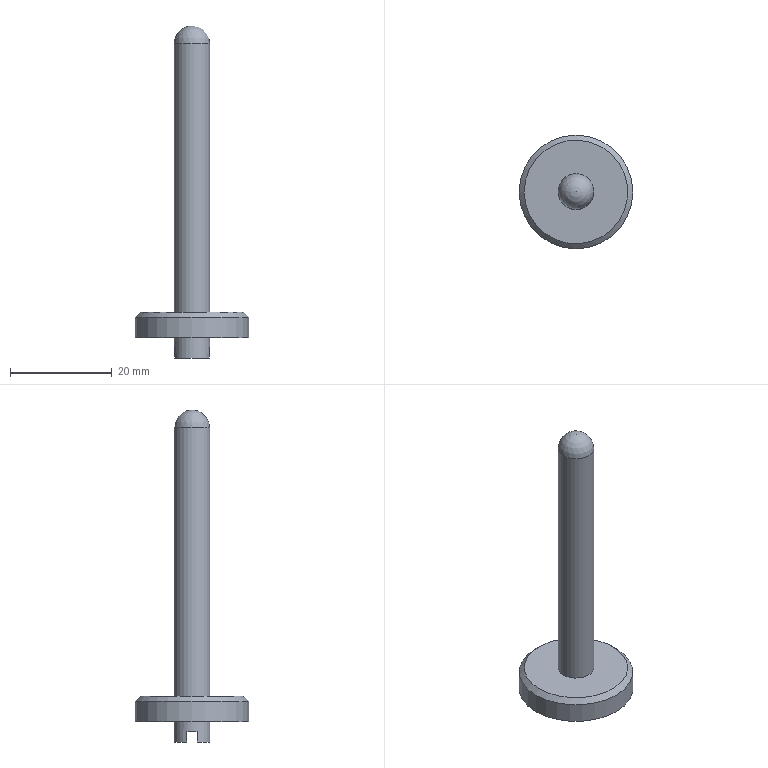Component | NX | VALVE_STEM | 1 solid | 12 faces | box 22.37 x 22.37 x 65.29 mm | volume 4179 mm3 | plane 7 | cylinder 3 | cone 1 | sphere 1 | commonest cylinder face diameters 7 x2 22.369 x1
STEP:
#1=CARTESIAN_POINT('',(0.,0.,0.));
#2=DIRECTION('',(0.,0.,1.));
#3=DIRECTION('',(1.,0.,0.));
#4=AXIS2_PLACEMENT_3D('',#1,#2,#3);
#5=CARTESIAN_POINT('',(-3.354,1.,34.567));
#6=VERTEX_POINT('',#5);
#7=CARTESIAN_POINT('',(3.354,1.,34.567));
#8=VERTEX_POINT('',#7);
#9=CARTESIAN_POINT('',(-8.45,1.,34.567));
#10=DIRECTION('',(1.,0.,0.));
#11=VECTOR('',#10,1.);
#12=LINE('',#9,#11);
#13=CARTESIAN_POINT('',(0.,0.,34.567));
#14=DIRECTION('',(0.,0.,-1.));
#15=DIRECTION('',(-1.,0.,0.));
#16=AXIS2_PLACEMENT_3D('',#13,#14,#15);
#17=PLANE('',#16);
#18=CARTESIAN_POINT('',(8.45,1.));
#19=DIRECTION('',(-1.,0.));
#20=VECTOR('',#19,1.);
#21=LINE('',#18,#20);
#22=(GEOMETRIC_REPRESENTATION_CONTEXT(2)PARAMETRIC_REPRESENTATION_CONTEXT()REPRESENTATION_CONTEXT('',''));
#23=DEFINITIONAL_REPRESENTATION('',(#21),#22);
#24=PCURVE('',#17,#23);
#25=CARTESIAN_POINT('',(-8.45,1.,36.567));
#26=DIRECTION('',(0.,1.,0.));
#27=DIRECTION('',(0.,0.,1.));
#28=AXIS2_PLACEMENT_3D('',#25,#26,#27);
#29=PLANE('',#28);
#30=CARTESIAN_POINT('',(-2.,0.));
#31=DIRECTION('',(0.,1.));
#32=VECTOR('',#31,1.);
#33=LINE('',#30,#32);
#34=(GEOMETRIC_REPRESENTATION_CONTEXT(2)PARAMETRIC_REPRESENTATION_CONTEXT()REPRESENTATION_CONTEXT('',''));
#35=DEFINITIONAL_REPRESENTATION('',(#33),#34);
#36=PCURVE('',#29,#35);
#37=SURFACE_CURVE('',#12,(#24,#36),.PCURVE_S1.);
#38=EDGE_CURVE('',#6,#8,#37,.T.);
#39=ORIENTED_EDGE('',*,*,#38,.F.);
#40=CARTESIAN_POINT('',(0.,0.,34.567));
#41=DIRECTION('',(0.,0.,-1.));
#42=DIRECTION('',(1.,0.,0.));
#43=AXIS2_PLACEMENT_3D('',#40,#41,#42);
#44=CIRCLE('',#43,3.5);
#45=CARTESIAN_POINT('',(0.,0.));
#46=DIRECTION('',(-1.,0.));
#47=AXIS2_PLACEMENT_2D('',#45,#46);
#48=CIRCLE('',#47,3.5);
#49=(GEOMETRIC_REPRESENTATION_CONTEXT(2)PARAMETRIC_REPRESENTATION_CONTEXT()REPRESENTATION_CONTEXT('',''));
#50=DEFINITIONAL_REPRESENTATION('',(#48),#49);
#51=PCURVE('',#17,#50);
#52=CARTESIAN_POINT('',(0.,0.,34.567));
#53=DIRECTION('',(0.,0.,1.));
#54=DIRECTION('',(1.,0.,0.));
#55=AXIS2_PLACEMENT_3D('',#52,#53,#54);
#56=CYLINDRICAL_SURFACE('',#55,3.5);
#57=CARTESIAN_POINT('',(6.283,0.));
#58=DIRECTION('',(-1.,0.));
#59=VECTOR('',#58,1.);
#60=LINE('',#57,#59);
#61=(GEOMETRIC_REPRESENTATION_CONTEXT(2)PARAMETRIC_REPRESENTATION_CONTEXT()REPRESENTATION_CONTEXT('',''));
#62=DEFINITIONAL_REPRESENTATION('',(#60),#61);
#63=PCURVE('',#56,#62);
#64=SURFACE_CURVE('',#44,(#51,#63),.PCURVE_S1.);
#65=EDGE_CURVE('',#6,#8,#64,.T.);
#66=ORIENTED_EDGE('',*,*,#65,.T.);
#67=EDGE_LOOP('',(#39,#66));
#68=FACE_BOUND('',#67,.T.);
#69=ADVANCED_FACE('',(#68),#17,.T.);
#70=CARTESIAN_POINT('',(3.5,0.,38.567));
#71=VERTEX_POINT('',#70);
#72=CARTESIAN_POINT('',(0.,0.,38.567));
#73=DIRECTION('',(0.,0.,-1.));
#74=DIRECTION('',(1.,0.,0.));
#75=AXIS2_PLACEMENT_3D('',#72,#73,#74);
#76=CIRCLE('',#75,3.5);
#77=CARTESIAN_POINT('',(0.,0.,38.567));
#78=DIRECTION('',(0.,0.,1.));
#79=DIRECTION('',(1.,0.,0.));
#80=AXIS2_PLACEMENT_3D('',#77,#78,#79);
#81=PLANE('',#80);
#82=CARTESIAN_POINT('',(3.5,-0.));
#83=CARTESIAN_POINT('',(3.5,-6.062));
#84=CARTESIAN_POINT('',(-1.75,-3.031));
#85=CARTESIAN_POINT('',(-7.,-0.));
#86=CARTESIAN_POINT('',(-1.75,3.031));
#87=CARTESIAN_POINT('',(3.5,6.062));
#88=CARTESIAN_POINT('',(3.5,-0.));
#89=(BOUNDED_CURVE()B_SPLINE_CURVE(2,(#82,#83,#84,#85,#86,#87,#88),.UNSPECIFIED.,.T.,.F.)B_SPLINE_CURVE_WITH_KNOTS((1,2,2,2,2,1),(-2.094,0.,2.094,4.189,6.283,8.378),.UNSPECIFIED.)CURVE()GEOMETRIC_REPRESENTATION_ITEM()RATIONAL_B_SPLINE_CURVE((1.,0.5,1.,0.5,1.,0.5,1.))REPRESENTATION_ITEM(''));
#90=(GEOMETRIC_REPRESENTATION_CONTEXT(2)PARAMETRIC_REPRESENTATION_CONTEXT()REPRESENTATION_CONTEXT('',''));
#91=DEFINITIONAL_REPRESENTATION('',(#89),#90);
#92=PCURVE('',#81,#91);
#93=CARTESIAN_POINT('',(6.283,4.));
#94=DIRECTION('',(-1.,0.));
#95=VECTOR('',#94,1.);
#96=LINE('',#93,#95);
#97=(GEOMETRIC_REPRESENTATION_CONTEXT(2)PARAMETRIC_REPRESENTATION_CONTEXT()REPRESENTATION_CONTEXT('',''));
#98=DEFINITIONAL_REPRESENTATION('',(#96),#97);
#99=PCURVE('',#56,#98);
#100=SURFACE_CURVE('',#76,(#92,#99),.PCURVE_S1.);
#101=EDGE_CURVE('',#71,#71,#100,.T.);
#102=ORIENTED_EDGE('',*,*,#101,.F.);
#103=EDGE_LOOP('',(#102));
#104=FACE_BOUND('',#103,.T.);
#105=CARTESIAN_POINT('',(11.184,0.,38.567));
#106=VERTEX_POINT('',#105);
#107=CARTESIAN_POINT('',(0.,0.,38.567));
#108=DIRECTION('',(0.,0.,1.));
#109=DIRECTION('',(1.,0.,0.));
#110=AXIS2_PLACEMENT_3D('',#107,#108,#109);
#111=CIRCLE('',#110,11.184);
#112=CARTESIAN_POINT('',(0.,-0.));
#113=DIRECTION('',(1.,0.));
#114=AXIS2_PLACEMENT_2D('',#112,#113);
#115=CIRCLE('',#114,11.184);
#116=(GEOMETRIC_REPRESENTATION_CONTEXT(2)PARAMETRIC_REPRESENTATION_CONTEXT()REPRESENTATION_CONTEXT('',''));
#117=DEFINITIONAL_REPRESENTATION('',(#115),#116);
#118=PCURVE('',#81,#117);
#119=CARTESIAN_POINT('',(0.,0.,79.857));
#120=DIRECTION('',(0.,0.,1.));
#121=DIRECTION('',(1.,0.,0.));
#122=AXIS2_PLACEMENT_3D('',#119,#120,#121);
#123=CYLINDRICAL_SURFACE('',#122,11.184);
#124=CARTESIAN_POINT('',(0.,-41.29));
#125=DIRECTION('',(1.,0.));
#126=VECTOR('',#125,1.);
#127=LINE('',#124,#126);
#128=(GEOMETRIC_REPRESENTATION_CONTEXT(2)PARAMETRIC_REPRESENTATION_CONTEXT()REPRESENTATION_CONTEXT('',''));
#129=DEFINITIONAL_REPRESENTATION('',(#127),#128);
#130=PCURVE('',#123,#129);
#131=SURFACE_CURVE('',#111,(#118,#130),.PCURVE_S1.);
#132=EDGE_CURVE('',#106,#106,#131,.T.);
#133=ORIENTED_EDGE('',*,*,#132,.F.);
#134=EDGE_LOOP('',(#133));
#135=FACE_BOUND('',#134,.T.);
#136=ADVANCED_FACE('',(#104,#135),#81,.F.);
#137=CARTESIAN_POINT('',(-11.184,0.,42.567));
#138=VERTEX_POINT('',#137);
#139=CARTESIAN_POINT('',(11.184,0.,42.567));
#140=VERTEX_POINT('',#139);
#141=CARTESIAN_POINT('',(0.,0.,42.567));
#142=DIRECTION('',(0.,0.,-1.));
#143=DIRECTION('',(-1.,0.,0.));
#144=AXIS2_PLACEMENT_3D('',#141,#142,#143);
#145=CIRCLE('',#144,11.184);
#146=CARTESIAN_POINT('',(3.142,-37.29));
#147=DIRECTION('',(-1.,0.));
#148=VECTOR('',#147,1.);
#149=LINE('',#146,#148);
#150=(GEOMETRIC_REPRESENTATION_CONTEXT(2)PARAMETRIC_REPRESENTATION_CONTEXT()REPRESENTATION_CONTEXT('',''));
#151=DEFINITIONAL_REPRESENTATION('',(#149),#150);
#152=PCURVE('',#123,#151);
#153=CARTESIAN_POINT('',(0.,0.,43.567));
#154=DIRECTION('',(0.,0.,-1.));
#155=DIRECTION('',(-1.,0.,0.));
#156=AXIS2_PLACEMENT_3D('',#153,#154,#155);
#157=CONICAL_SURFACE('',#156,10.184,0.7854);
#158=CARTESIAN_POINT('',(0.,1.));
#159=DIRECTION('',(1.,0.));
#160=VECTOR('',#159,1.);
#161=LINE('',#158,#160);
#162=(GEOMETRIC_REPRESENTATION_CONTEXT(2)PARAMETRIC_REPRESENTATION_CONTEXT()REPRESENTATION_CONTEXT('',''));
#163=DEFINITIONAL_REPRESENTATION('',(#161),#162);
#164=PCURVE('',#157,#163);
#165=SURFACE_CURVE('',#145,(#152,#164),.PCURVE_S1.);
#166=EDGE_CURVE('',#138,#140,#165,.T.);
#167=ORIENTED_EDGE('',*,*,#166,.T.);
#168=CARTESIAN_POINT('',(11.184,-0.,38.567));
#169=CARTESIAN_POINT('',(11.184,-0.,42.567));
#170=B_SPLINE_CURVE_WITH_KNOTS('',1,(#168,#169),.UNSPECIFIED.,.F.,.F.,(2,2),(-41.29,-37.29),.PIECEWISE_BEZIER_KNOTS.);
#171=CARTESIAN_POINT('',(0.,0.));
#172=DIRECTION('',(0.,1.));
#173=VECTOR('',#172,1.);
#174=LINE('',#171,#173);
#175=(GEOMETRIC_REPRESENTATION_CONTEXT(2)PARAMETRIC_REPRESENTATION_CONTEXT()REPRESENTATION_CONTEXT('',''));
#176=DEFINITIONAL_REPRESENTATION('',(#174),#175);
#177=PCURVE('',#123,#176);
#178=CARTESIAN_POINT('',(6.283,0.));
#179=DIRECTION('',(0.,1.));
#180=VECTOR('',#179,1.);
#181=LINE('',#178,#180);
#182=(GEOMETRIC_REPRESENTATION_CONTEXT(2)PARAMETRIC_REPRESENTATION_CONTEXT()REPRESENTATION_CONTEXT('',''));
#183=DEFINITIONAL_REPRESENTATION('',(#181),#182);
#184=PCURVE('',#123,#183);
#185=SEAM_CURVE('',#170,(#177,#184),.PCURVE_S1.);
#186=EDGE_CURVE('',#106,#140,#185,.T.);
#187=ORIENTED_EDGE('',*,*,#186,.F.);
#188=ORIENTED_EDGE('',*,*,#132,.T.);
#189=ORIENTED_EDGE('',*,*,#186,.T.);
#190=CARTESIAN_POINT('',(0.,0.,42.567));
#191=DIRECTION('',(0.,0.,-1.));
#192=DIRECTION('',(-1.,0.,0.));
#193=AXIS2_PLACEMENT_3D('',#190,#191,#192);
#194=CIRCLE('',#193,11.184);
#195=CARTESIAN_POINT('',(9.425,-37.29));
#196=DIRECTION('',(-1.,0.));
#197=VECTOR('',#196,1.);
#198=LINE('',#195,#197);
#199=(GEOMETRIC_REPRESENTATION_CONTEXT(2)PARAMETRIC_REPRESENTATION_CONTEXT()REPRESENTATION_CONTEXT('',''));
#200=DEFINITIONAL_REPRESENTATION('',(#198),#199);
#201=PCURVE('',#123,#200);
#202=CARTESIAN_POINT('',(0.,1.));
#203=DIRECTION('',(1.,0.));
#204=VECTOR('',#203,1.);
#205=LINE('',#202,#204);
#206=(GEOMETRIC_REPRESENTATION_CONTEXT(2)PARAMETRIC_REPRESENTATION_CONTEXT()REPRESENTATION_CONTEXT('',''));
#207=DEFINITIONAL_REPRESENTATION('',(#205),#206);
#208=PCURVE('',#157,#207);
#209=SURFACE_CURVE('',#194,(#201,#208),.PCURVE_S1.);
#210=EDGE_CURVE('',#140,#138,#209,.T.);
#211=ORIENTED_EDGE('',*,*,#210,.T.);
#212=EDGE_LOOP('',(#167,#187,#188,#189,#211));
#213=FACE_BOUND('',#212,.T.);
#214=ADVANCED_FACE('',(#213),#123,.T.);
#215=CARTESIAN_POINT('',(-10.184,0.,43.567));
#216=VERTEX_POINT('',#215);
#217=CARTESIAN_POINT('',(0.,0.,43.567));
#218=DIRECTION('',(0.,0.,1.));
#219=DIRECTION('',(-1.,0.,0.));
#220=AXIS2_PLACEMENT_3D('',#217,#218,#219);
#221=CIRCLE('',#220,10.184);
#222=CARTESIAN_POINT('',(0.,11.184,43.567));
#223=DIRECTION('',(0.,0.,-1.));
#224=DIRECTION('',(-1.,0.,0.));
#225=AXIS2_PLACEMENT_3D('',#222,#223,#224);
#226=PLANE('',#225);
#227=CARTESIAN_POINT('',(10.184,-11.184));
#228=CARTESIAN_POINT('',(10.184,-28.824));
#229=CARTESIAN_POINT('',(-5.092,-20.004));
#230=CARTESIAN_POINT('',(-20.369,-11.184));
#231=CARTESIAN_POINT('',(-5.092,-2.364));
#232=CARTESIAN_POINT('',(10.184,6.455));
#233=CARTESIAN_POINT('',(10.184,-11.184));
#234=(BOUNDED_CURVE()B_SPLINE_CURVE(2,(#227,#228,#229,#230,#231,#232,#233),.UNSPECIFIED.,.T.,.F.)B_SPLINE_CURVE_WITH_KNOTS((1,2,2,2,2,1),(-2.094,0.,2.094,4.189,6.283,8.378),.UNSPECIFIED.)CURVE()GEOMETRIC_REPRESENTATION_ITEM()RATIONAL_B_SPLINE_CURVE((1.,0.5,1.,0.5,1.,0.5,1.))REPRESENTATION_ITEM(''));
#235=(GEOMETRIC_REPRESENTATION_CONTEXT(2)PARAMETRIC_REPRESENTATION_CONTEXT()REPRESENTATION_CONTEXT('',''));
#236=DEFINITIONAL_REPRESENTATION('',(#234),#235);
#237=PCURVE('',#226,#236);
#238=CARTESIAN_POINT('',(6.283,0.));
#239=DIRECTION('',(-1.,0.));
#240=VECTOR('',#239,1.);
#241=LINE('',#238,#240);
#242=(GEOMETRIC_REPRESENTATION_CONTEXT(2)PARAMETRIC_REPRESENTATION_CONTEXT()REPRESENTATION_CONTEXT('',''));
#243=DEFINITIONAL_REPRESENTATION('',(#241),#242);
#244=PCURVE('',#157,#243);
#245=SURFACE_CURVE('',#221,(#237,#244),.PCURVE_S1.);
#246=EDGE_CURVE('',#216,#216,#245,.T.);
#247=ORIENTED_EDGE('',*,*,#246,.T.);
#248=EDGE_LOOP('',(#247));
#249=FACE_BOUND('',#248,.T.);
#250=CARTESIAN_POINT('',(3.5,0.,43.567));
#251=VERTEX_POINT('',#250);
#252=CARTESIAN_POINT('',(0.,0.,43.567));
#253=DIRECTION('',(0.,0.,1.));
#254=DIRECTION('',(1.,0.,0.));
#255=AXIS2_PLACEMENT_3D('',#252,#253,#254);
#256=CIRCLE('',#255,3.5);
#257=CARTESIAN_POINT('',(-3.5,-11.184));
#258=CARTESIAN_POINT('',(-3.5,-5.122));
#259=CARTESIAN_POINT('',(1.75,-8.153));
#260=CARTESIAN_POINT('',(7.,-11.184));
#261=CARTESIAN_POINT('',(1.75,-14.215));
#262=CARTESIAN_POINT('',(-3.5,-17.246));
#263=CARTESIAN_POINT('',(-3.5,-11.184));
#264=(BOUNDED_CURVE()B_SPLINE_CURVE(2,(#257,#258,#259,#260,#261,#262,#263),.UNSPECIFIED.,.T.,.F.)B_SPLINE_CURVE_WITH_KNOTS((1,2,2,2,2,1),(-2.094,0.,2.094,4.189,6.283,8.378),.UNSPECIFIED.)CURVE()GEOMETRIC_REPRESENTATION_ITEM()RATIONAL_B_SPLINE_CURVE((1.,0.5,1.,0.5,1.,0.5,1.))REPRESENTATION_ITEM(''));
#265=(GEOMETRIC_REPRESENTATION_CONTEXT(2)PARAMETRIC_REPRESENTATION_CONTEXT()REPRESENTATION_CONTEXT('',''));
#266=DEFINITIONAL_REPRESENTATION('',(#264),#265);
#267=PCURVE('',#226,#266);
#268=CARTESIAN_POINT('',(0.,0.,79.857));
#269=DIRECTION('',(0.,0.,1.));
#270=DIRECTION('',(1.,0.,0.));
#271=AXIS2_PLACEMENT_3D('',#268,#269,#270);
#272=CYLINDRICAL_SURFACE('',#271,3.5);
#273=CARTESIAN_POINT('',(0.,-36.29));
#274=DIRECTION('',(1.,0.));
#275=VECTOR('',#274,1.);
#276=LINE('',#273,#275);
#277=(GEOMETRIC_REPRESENTATION_CONTEXT(2)PARAMETRIC_REPRESENTATION_CONTEXT()REPRESENTATION_CONTEXT('',''));
#278=DEFINITIONAL_REPRESENTATION('',(#276),#277);
#279=PCURVE('',#272,#278);
#280=SURFACE_CURVE('',#256,(#267,#279),.PCURVE_S1.);
#281=EDGE_CURVE('',#251,#251,#280,.T.);
#282=ORIENTED_EDGE('',*,*,#281,.F.);
#283=EDGE_LOOP('',(#282));
#284=FACE_BOUND('',#283,.T.);
#285=ADVANCED_FACE('',(#249,#284),#226,.F.);
#286=CARTESIAN_POINT('',(3.5,0.,96.357));
#287=VERTEX_POINT('',#286);
#288=CARTESIAN_POINT('',(-3.5,0.,96.357));
#289=VERTEX_POINT('',#288);
#290=CARTESIAN_POINT('',(0.,0.,96.357));
#291=DIRECTION('',(0.,0.,-1.));
#292=DIRECTION('',(1.,0.,0.));
#293=AXIS2_PLACEMENT_3D('',#290,#291,#292);
#294=CIRCLE('',#293,3.5);
#295=CARTESIAN_POINT('',(6.283,16.5));
#296=DIRECTION('',(-1.,0.));
#297=VECTOR('',#296,1.);
#298=LINE('',#295,#297);
#299=(GEOMETRIC_REPRESENTATION_CONTEXT(2)PARAMETRIC_REPRESENTATION_CONTEXT()REPRESENTATION_CONTEXT('',''));
#300=DEFINITIONAL_REPRESENTATION('',(#298),#299);
#301=PCURVE('',#272,#300);
#302=CARTESIAN_POINT('',(0.,0.,96.357));
#303=DIRECTION('',(-0.,0.,-1.));
#304=DIRECTION('',(-1.,0.,0.));
#305=AXIS2_PLACEMENT_3D('',#302,#303,#304);
#306=SPHERICAL_SURFACE('',#305,3.5);
#307=CARTESIAN_POINT('',(3.142,0.));
#308=CARTESIAN_POINT('',(3.237,0.));
#309=CARTESIAN_POINT('',(3.427,0.));
#310=CARTESIAN_POINT('',(3.713,0.));
#311=CARTESIAN_POINT('',(3.998,0.));
#312=CARTESIAN_POINT('',(4.284,0.));
#313=CARTESIAN_POINT('',(4.57,0.));
#314=CARTESIAN_POINT('',(4.855,0.));
#315=CARTESIAN_POINT('',(5.141,0.));
#316=CARTESIAN_POINT('',(5.426,0.));
#317=CARTESIAN_POINT('',(5.712,0.));
#318=CARTESIAN_POINT('',(5.998,0.));
#319=CARTESIAN_POINT('',(6.283,0.));
#320=CARTESIAN_POINT('',(6.569,0.));
#321=CARTESIAN_POINT('',(6.854,0.));
#322=CARTESIAN_POINT('',(7.14,0.));
#323=CARTESIAN_POINT('',(7.426,0.));
#324=CARTESIAN_POINT('',(7.711,0.));
#325=CARTESIAN_POINT('',(7.997,0.));
#326=CARTESIAN_POINT('',(8.282,0.));
#327=CARTESIAN_POINT('',(8.568,0.));
#328=CARTESIAN_POINT('',(8.854,0.));
#329=CARTESIAN_POINT('',(9.139,0.));
#330=CARTESIAN_POINT('',(9.33,0.));
#331=CARTESIAN_POINT('',(9.425,0.));
#332=B_SPLINE_CURVE_WITH_KNOTS('',3,(#307,#308,#309,#310,#311,#312,#313,#314,#315,#316,#317,#318,#319,#320,#321,#322,#323,#324,#325,#326,#327,#328,#329,#330,#331),.UNSPECIFIED.,.F.,.F.,(4,1,1,1,1,1,1,1,1,1,1,1,1,1,1,1,1,1,1,1,1,1,4),(0.,0.2856,0.5712,0.8568,1.142,1.428,1.714,1.999,2.285,2.57,2.856,3.142,3.427,3.713,3.998,4.284,4.57,4.855,5.141,5.426,5.712,5.998,6.283),.QUASI_UNIFORM_KNOTS.);
#333=(GEOMETRIC_REPRESENTATION_CONTEXT(2)PARAMETRIC_REPRESENTATION_CONTEXT()REPRESENTATION_CONTEXT('',''));
#334=DEFINITIONAL_REPRESENTATION('',(#332),#333);
#335=PCURVE('',#306,#334);
#336=SURFACE_CURVE('',#294,(#301,#335),.PCURVE_S1.);
#337=EDGE_CURVE('',#287,#289,#336,.T.);
#338=ORIENTED_EDGE('',*,*,#337,.T.);
#339=CARTESIAN_POINT('',(0.,0.,96.357));
#340=DIRECTION('',(0.,0.,-1.));
#341=DIRECTION('',(1.,0.,0.));
#342=AXIS2_PLACEMENT_3D('',#339,#340,#341);
#343=CIRCLE('',#342,3.5);
#344=CARTESIAN_POINT('',(6.283,16.5));
#345=DIRECTION('',(-1.,0.));
#346=VECTOR('',#345,1.);
#347=LINE('',#344,#346);
#348=(GEOMETRIC_REPRESENTATION_CONTEXT(2)PARAMETRIC_REPRESENTATION_CONTEXT()REPRESENTATION_CONTEXT('',''));
#349=DEFINITIONAL_REPRESENTATION('',(#347),#348);
#350=PCURVE('',#272,#349);
#351=CARTESIAN_POINT('',(-3.142,0.));
#352=CARTESIAN_POINT('',(-3.046,0.));
#353=CARTESIAN_POINT('',(-2.856,0.));
#354=CARTESIAN_POINT('',(-2.57,0.));
#355=CARTESIAN_POINT('',(-2.285,0.));
#356=CARTESIAN_POINT('',(-1.999,0.));
#357=CARTESIAN_POINT('',(-1.714,0.));
#358=CARTESIAN_POINT('',(-1.428,0.));
#359=CARTESIAN_POINT('',(-1.142,0.));
#360=CARTESIAN_POINT('',(-0.8568,0.));
#361=CARTESIAN_POINT('',(-0.5712,0.));
#362=CARTESIAN_POINT('',(-0.2856,0.));
#363=CARTESIAN_POINT('',(0.,0.));
#364=CARTESIAN_POINT('',(0.2856,0.));
#365=CARTESIAN_POINT('',(0.5712,0.));
#366=CARTESIAN_POINT('',(0.8568,0.));
#367=CARTESIAN_POINT('',(1.142,0.));
#368=CARTESIAN_POINT('',(1.428,0.));
#369=CARTESIAN_POINT('',(1.714,0.));
#370=CARTESIAN_POINT('',(1.999,0.));
#371=CARTESIAN_POINT('',(2.285,0.));
#372=CARTESIAN_POINT('',(2.57,0.));
#373=CARTESIAN_POINT('',(2.856,0.));
#374=CARTESIAN_POINT('',(3.046,0.));
#375=CARTESIAN_POINT('',(3.142,0.));
#376=B_SPLINE_CURVE_WITH_KNOTS('',3,(#351,#352,#353,#354,#355,#356,#357,#358,#359,#360,#361,#362,#363,#364,#365,#366,#367,#368,#369,#370,#371,#372,#373,#374,#375),.UNSPECIFIED.,.F.,.F.,(4,1,1,1,1,1,1,1,1,1,1,1,1,1,1,1,1,1,1,1,1,1,4),(0.,0.2856,0.5712,0.8568,1.142,1.428,1.714,1.999,2.285,2.57,2.856,3.142,3.427,3.713,3.998,4.284,4.57,4.855,5.141,5.426,5.712,5.998,6.283),.QUASI_UNIFORM_KNOTS.);
#377=(GEOMETRIC_REPRESENTATION_CONTEXT(2)PARAMETRIC_REPRESENTATION_CONTEXT()REPRESENTATION_CONTEXT('',''));
#378=DEFINITIONAL_REPRESENTATION('',(#376),#377);
#379=PCURVE('',#306,#378);
#380=SURFACE_CURVE('',#343,(#350,#379),.PCURVE_S1.);
#381=EDGE_CURVE('',#289,#287,#380,.T.);
#382=ORIENTED_EDGE('',*,*,#381,.T.);
#383=CARTESIAN_POINT('',(3.5,-0.,43.567));
#384=CARTESIAN_POINT('',(3.5,-0.,96.357));
#385=B_SPLINE_CURVE_WITH_KNOTS('',1,(#383,#384),.UNSPECIFIED.,.F.,.F.,(2,2),(-36.29,16.5),.PIECEWISE_BEZIER_KNOTS.);
#386=CARTESIAN_POINT('',(0.,0.));
#387=DIRECTION('',(0.,1.));
#388=VECTOR('',#387,1.);
#389=LINE('',#386,#388);
#390=(GEOMETRIC_REPRESENTATION_CONTEXT(2)PARAMETRIC_REPRESENTATION_CONTEXT()REPRESENTATION_CONTEXT('',''));
#391=DEFINITIONAL_REPRESENTATION('',(#389),#390);
#392=PCURVE('',#272,#391);
#393=CARTESIAN_POINT('',(6.283,0.));
#394=DIRECTION('',(0.,1.));
#395=VECTOR('',#394,1.);
#396=LINE('',#393,#395);
#397=(GEOMETRIC_REPRESENTATION_CONTEXT(2)PARAMETRIC_REPRESENTATION_CONTEXT()REPRESENTATION_CONTEXT('',''));
#398=DEFINITIONAL_REPRESENTATION('',(#396),#397);
#399=PCURVE('',#272,#398);
#400=SEAM_CURVE('',#385,(#392,#399),.PCURVE_S1.);
#401=EDGE_CURVE('',#251,#287,#400,.T.);
#402=ORIENTED_EDGE('',*,*,#401,.F.);
#403=ORIENTED_EDGE('',*,*,#281,.T.);
#404=ORIENTED_EDGE('',*,*,#401,.T.);
#405=EDGE_LOOP('',(#338,#382,#402,#403,#404));
#406=FACE_BOUND('',#405,.T.);
#407=ADVANCED_FACE('',(#406),#272,.T.);
#408=ORIENTED_EDGE('',*,*,#166,.F.);
#409=CARTESIAN_POINT('',(-10.184,-0.,43.567));
#410=CARTESIAN_POINT('',(-11.184,-0.,42.567));
#411=B_SPLINE_CURVE_WITH_KNOTS('',1,(#409,#410),.UNSPECIFIED.,.F.,.F.,(2,2),(0.,1.414),.PIECEWISE_BEZIER_KNOTS.);
#412=CARTESIAN_POINT('',(0.,0.));
#413=DIRECTION('',(0.,1.));
#414=VECTOR('',#413,1.);
#415=LINE('',#412,#414);
#416=(GEOMETRIC_REPRESENTATION_CONTEXT(2)PARAMETRIC_REPRESENTATION_CONTEXT()REPRESENTATION_CONTEXT('',''));
#417=DEFINITIONAL_REPRESENTATION('',(#415),#416);
#418=PCURVE('',#157,#417);
#419=CARTESIAN_POINT('',(6.283,0.));
#420=DIRECTION('',(0.,1.));
#421=VECTOR('',#420,1.);
#422=LINE('',#419,#421);
#423=(GEOMETRIC_REPRESENTATION_CONTEXT(2)PARAMETRIC_REPRESENTATION_CONTEXT()REPRESENTATION_CONTEXT('',''));
#424=DEFINITIONAL_REPRESENTATION('',(#422),#423);
#425=PCURVE('',#157,#424);
#426=SEAM_CURVE('',#411,(#418,#425),.PCURVE_S1.);
#427=EDGE_CURVE('',#216,#138,#426,.T.);
#428=ORIENTED_EDGE('',*,*,#427,.F.);
#429=ORIENTED_EDGE('',*,*,#246,.F.);
#430=ORIENTED_EDGE('',*,*,#427,.T.);
#431=ORIENTED_EDGE('',*,*,#210,.F.);
#432=EDGE_LOOP('',(#408,#428,#429,#430,#431));
#433=FACE_BOUND('',#432,.T.);
#434=ADVANCED_FACE('',(#433),#157,.T.);
#435=CARTESIAN_POINT('',(3.5,0.,36.567));
#436=VERTEX_POINT('',#435);
#437=CARTESIAN_POINT('',(3.354,-1.,36.567));
#438=VERTEX_POINT('',#437);
#439=CARTESIAN_POINT('',(0.,0.,36.567));
#440=DIRECTION('',(0.,0.,-1.));
#441=DIRECTION('',(-1.,0.,0.));
#442=AXIS2_PLACEMENT_3D('',#439,#440,#441);
#443=CIRCLE('',#442,3.5);
#444=CARTESIAN_POINT('',(9.425,2.));
#445=DIRECTION('',(-1.,0.));
#446=VECTOR('',#445,1.);
#447=LINE('',#444,#446);
#448=(GEOMETRIC_REPRESENTATION_CONTEXT(2)PARAMETRIC_REPRESENTATION_CONTEXT()REPRESENTATION_CONTEXT('',''));
#449=DEFINITIONAL_REPRESENTATION('',(#447),#448);
#450=PCURVE('',#56,#449);
#451=CARTESIAN_POINT('',(0.,0.,36.567));
#452=DIRECTION('',(0.,0.,-1.));
#453=DIRECTION('',(-1.,0.,0.));
#454=AXIS2_PLACEMENT_3D('',#451,#452,#453);
#455=PLANE('',#454);
#456=CARTESIAN_POINT('',(0.,0.));
#457=DIRECTION('',(1.,0.));
#458=AXIS2_PLACEMENT_2D('',#456,#457);
#459=CIRCLE('',#458,3.5);
#460=(GEOMETRIC_REPRESENTATION_CONTEXT(2)PARAMETRIC_REPRESENTATION_CONTEXT()REPRESENTATION_CONTEXT('',''));
#461=DEFINITIONAL_REPRESENTATION('',(#459),#460);
#462=PCURVE('',#455,#461);
#463=SURFACE_CURVE('',#443,(#450,#462),.PCURVE_S1.);
#464=EDGE_CURVE('',#436,#438,#463,.T.);
#465=ORIENTED_EDGE('',*,*,#464,.F.);
#466=CARTESIAN_POINT('',(3.5,0.,36.567));
#467=CARTESIAN_POINT('',(3.5,0.,38.567));
#468=B_SPLINE_CURVE_WITH_KNOTS('',1,(#466,#467),.UNSPECIFIED.,.F.,.F.,(2,2),(2.,4.),.PIECEWISE_BEZIER_KNOTS.);
#469=CARTESIAN_POINT('',(6.283,0.));
#470=DIRECTION('',(0.,1.));
#471=VECTOR('',#470,1.);
#472=LINE('',#469,#471);
#473=(GEOMETRIC_REPRESENTATION_CONTEXT(2)PARAMETRIC_REPRESENTATION_CONTEXT()REPRESENTATION_CONTEXT('',''));
#474=DEFINITIONAL_REPRESENTATION('',(#472),#473);
#475=PCURVE('',#56,#474);
#476=CARTESIAN_POINT('',(0.,0.));
#477=DIRECTION('',(0.,1.));
#478=VECTOR('',#477,1.);
#479=LINE('',#476,#478);
#480=(GEOMETRIC_REPRESENTATION_CONTEXT(2)PARAMETRIC_REPRESENTATION_CONTEXT()REPRESENTATION_CONTEXT('',''));
#481=DEFINITIONAL_REPRESENTATION('',(#479),#480);
#482=PCURVE('',#56,#481);
#483=SEAM_CURVE('',#468,(#475,#482),.PCURVE_S1.);
#484=EDGE_CURVE('',#436,#71,#483,.T.);
#485=ORIENTED_EDGE('',*,*,#484,.T.);
#486=ORIENTED_EDGE('',*,*,#101,.T.);
#487=ORIENTED_EDGE('',*,*,#484,.F.);
#488=CARTESIAN_POINT('',(3.354,1.,36.567));
#489=VERTEX_POINT('',#488);
#490=CARTESIAN_POINT('',(0.,0.,36.567));
#491=DIRECTION('',(0.,0.,-1.));
#492=DIRECTION('',(-1.,0.,0.));
#493=AXIS2_PLACEMENT_3D('',#490,#491,#492);
#494=CIRCLE('',#493,3.5);
#495=CARTESIAN_POINT('',(3.142,2.));
#496=DIRECTION('',(-1.,0.));
#497=VECTOR('',#496,1.);
#498=LINE('',#495,#497);
#499=(GEOMETRIC_REPRESENTATION_CONTEXT(2)PARAMETRIC_REPRESENTATION_CONTEXT()REPRESENTATION_CONTEXT('',''));
#500=DEFINITIONAL_REPRESENTATION('',(#498),#499);
#501=PCURVE('',#56,#500);
#502=CARTESIAN_POINT('',(0.,0.));
#503=DIRECTION('',(1.,0.));
#504=AXIS2_PLACEMENT_2D('',#502,#503);
#505=CIRCLE('',#504,3.5);
#506=(GEOMETRIC_REPRESENTATION_CONTEXT(2)PARAMETRIC_REPRESENTATION_CONTEXT()REPRESENTATION_CONTEXT('',''));
#507=DEFINITIONAL_REPRESENTATION('',(#505),#506);
#508=PCURVE('',#455,#507);
#509=SURFACE_CURVE('',#494,(#501,#508),.PCURVE_S1.);
#510=EDGE_CURVE('',#489,#436,#509,.T.);
#511=ORIENTED_EDGE('',*,*,#510,.F.);
#512=CARTESIAN_POINT('',(3.354,1.,34.567));
#513=DIRECTION('',(0.,0.,-1.));
#514=VECTOR('',#513,1.);
#515=LINE('',#512,#514);
#516=CARTESIAN_POINT('',(0.2898,0.));
#517=DIRECTION('',(0.,-1.));
#518=VECTOR('',#517,1.);
#519=LINE('',#516,#518);
#520=(GEOMETRIC_REPRESENTATION_CONTEXT(2)PARAMETRIC_REPRESENTATION_CONTEXT()REPRESENTATION_CONTEXT('',''));
#521=DEFINITIONAL_REPRESENTATION('',(#519),#520);
#522=PCURVE('',#56,#521);
#523=CARTESIAN_POINT('',(-2.,11.804));
#524=DIRECTION('',(-1.,0.));
#525=VECTOR('',#524,1.);
#526=LINE('',#523,#525);
#527=(GEOMETRIC_REPRESENTATION_CONTEXT(2)PARAMETRIC_REPRESENTATION_CONTEXT()REPRESENTATION_CONTEXT('',''));
#528=DEFINITIONAL_REPRESENTATION('',(#526),#527);
#529=PCURVE('',#29,#528);
#530=SURFACE_CURVE('',#515,(#522,#529),.PCURVE_S1.);
#531=EDGE_CURVE('',#489,#8,#530,.T.);
#532=ORIENTED_EDGE('',*,*,#531,.T.);
#533=ORIENTED_EDGE('',*,*,#65,.F.);
#534=CARTESIAN_POINT('',(-3.354,1.,36.567));
#535=VERTEX_POINT('',#534);
#536=CARTESIAN_POINT('',(-3.354,1.,34.567));
#537=DIRECTION('',(0.,0.,1.));
#538=VECTOR('',#537,1.);
#539=LINE('',#536,#538);
#540=CARTESIAN_POINT('',(2.852,0.));
#541=DIRECTION('',(0.,1.));
#542=VECTOR('',#541,1.);
#543=LINE('',#540,#542);
#544=(GEOMETRIC_REPRESENTATION_CONTEXT(2)PARAMETRIC_REPRESENTATION_CONTEXT()REPRESENTATION_CONTEXT('',''));
#545=DEFINITIONAL_REPRESENTATION('',(#543),#544);
#546=PCURVE('',#56,#545);
#547=CARTESIAN_POINT('',(-2.,5.096));
#548=DIRECTION('',(1.,0.));
#549=VECTOR('',#548,1.);
#550=LINE('',#547,#549);
#551=(GEOMETRIC_REPRESENTATION_CONTEXT(2)PARAMETRIC_REPRESENTATION_CONTEXT()REPRESENTATION_CONTEXT('',''));
#552=DEFINITIONAL_REPRESENTATION('',(#550),#551);
#553=PCURVE('',#29,#552);
#554=SURFACE_CURVE('',#539,(#546,#553),.PCURVE_S1.);
#555=EDGE_CURVE('',#6,#535,#554,.T.);
#556=ORIENTED_EDGE('',*,*,#555,.T.);
#557=CARTESIAN_POINT('',(-3.354,-1.,36.567));
#558=VERTEX_POINT('',#557);
#559=CARTESIAN_POINT('',(0.,0.,36.567));
#560=DIRECTION('',(0.,0.,-1.));
#561=DIRECTION('',(-1.,0.,0.));
#562=AXIS2_PLACEMENT_3D('',#559,#560,#561);
#563=CIRCLE('',#562,3.5);
#564=CARTESIAN_POINT('',(9.425,2.));
#565=DIRECTION('',(-1.,0.));
#566=VECTOR('',#565,1.);
#567=LINE('',#564,#566);
#568=(GEOMETRIC_REPRESENTATION_CONTEXT(2)PARAMETRIC_REPRESENTATION_CONTEXT()REPRESENTATION_CONTEXT('',''));
#569=DEFINITIONAL_REPRESENTATION('',(#567),#568);
#570=PCURVE('',#56,#569);
#571=CARTESIAN_POINT('',(0.,0.));
#572=DIRECTION('',(1.,0.));
#573=AXIS2_PLACEMENT_2D('',#571,#572);
#574=CIRCLE('',#573,3.5);
#575=(GEOMETRIC_REPRESENTATION_CONTEXT(2)PARAMETRIC_REPRESENTATION_CONTEXT()REPRESENTATION_CONTEXT('',''));
#576=DEFINITIONAL_REPRESENTATION('',(#574),#575);
#577=PCURVE('',#455,#576);
#578=SURFACE_CURVE('',#563,(#570,#577),.PCURVE_S1.);
#579=EDGE_CURVE('',#558,#535,#578,.T.);
#580=ORIENTED_EDGE('',*,*,#579,.F.);
#581=CARTESIAN_POINT('',(-3.354,-1.,34.567));
#582=VERTEX_POINT('',#581);
#583=CARTESIAN_POINT('',(-3.354,-1.,34.567));
#584=DIRECTION('',(0.,0.,-1.));
#585=VECTOR('',#584,1.);
#586=LINE('',#583,#585);
#587=CARTESIAN_POINT('',(3.431,0.));
#588=DIRECTION('',(0.,-1.));
#589=VECTOR('',#588,1.);
#590=LINE('',#587,#589);
#591=(GEOMETRIC_REPRESENTATION_CONTEXT(2)PARAMETRIC_REPRESENTATION_CONTEXT()REPRESENTATION_CONTEXT('',''));
#592=DEFINITIONAL_REPRESENTATION('',(#590),#591);
#593=PCURVE('',#56,#592);
#594=CARTESIAN_POINT('',(8.45,-1.,36.567));
#595=DIRECTION('',(0.,-1.,0.));
#596=DIRECTION('',(0.,0.,-1.));
#597=AXIS2_PLACEMENT_3D('',#594,#595,#596);
#598=PLANE('',#597);
#599=CARTESIAN_POINT('',(2.,-11.804));
#600=DIRECTION('',(1.,0.));
#601=VECTOR('',#600,1.);
#602=LINE('',#599,#601);
#603=(GEOMETRIC_REPRESENTATION_CONTEXT(2)PARAMETRIC_REPRESENTATION_CONTEXT()REPRESENTATION_CONTEXT('',''));
#604=DEFINITIONAL_REPRESENTATION('',(#602),#603);
#605=PCURVE('',#598,#604);
#606=SURFACE_CURVE('',#586,(#593,#605),.PCURVE_S1.);
#607=EDGE_CURVE('',#558,#582,#606,.T.);
#608=ORIENTED_EDGE('',*,*,#607,.T.);
#609=CARTESIAN_POINT('',(3.354,-1.,34.567));
#610=VERTEX_POINT('',#609);
#611=CARTESIAN_POINT('',(0.,0.,34.567));
#612=DIRECTION('',(0.,0.,-1.));
#613=DIRECTION('',(1.,0.,0.));
#614=AXIS2_PLACEMENT_3D('',#611,#612,#613);
#615=CIRCLE('',#614,3.5);
#616=CARTESIAN_POINT('',(6.283,0.));
#617=DIRECTION('',(-1.,0.));
#618=VECTOR('',#617,1.);
#619=LINE('',#616,#618);
#620=(GEOMETRIC_REPRESENTATION_CONTEXT(2)PARAMETRIC_REPRESENTATION_CONTEXT()REPRESENTATION_CONTEXT('',''));
#621=DEFINITIONAL_REPRESENTATION('',(#619),#620);
#622=PCURVE('',#56,#621);
#623=CARTESIAN_POINT('',(0.,0.,34.567));
#624=DIRECTION('',(0.,0.,-1.));
#625=DIRECTION('',(-1.,0.,0.));
#626=AXIS2_PLACEMENT_3D('',#623,#624,#625);
#627=PLANE('',#626);
#628=CARTESIAN_POINT('',(0.,0.));
#629=DIRECTION('',(-1.,0.));
#630=AXIS2_PLACEMENT_2D('',#628,#629);
#631=CIRCLE('',#630,3.5);
#632=(GEOMETRIC_REPRESENTATION_CONTEXT(2)PARAMETRIC_REPRESENTATION_CONTEXT()REPRESENTATION_CONTEXT('',''));
#633=DEFINITIONAL_REPRESENTATION('',(#631),#632);
#634=PCURVE('',#627,#633);
#635=SURFACE_CURVE('',#615,(#622,#634),.PCURVE_S1.);
#636=EDGE_CURVE('',#610,#582,#635,.T.);
#637=ORIENTED_EDGE('',*,*,#636,.F.);
#638=CARTESIAN_POINT('',(3.354,-1.,34.567));
#639=DIRECTION('',(0.,0.,1.));
#640=VECTOR('',#639,1.);
#641=LINE('',#638,#640);
#642=CARTESIAN_POINT('',(5.993,0.));
#643=DIRECTION('',(0.,1.));
#644=VECTOR('',#643,1.);
#645=LINE('',#642,#644);
#646=(GEOMETRIC_REPRESENTATION_CONTEXT(2)PARAMETRIC_REPRESENTATION_CONTEXT()REPRESENTATION_CONTEXT('',''));
#647=DEFINITIONAL_REPRESENTATION('',(#645),#646);
#648=PCURVE('',#56,#647);
#649=CARTESIAN_POINT('',(2.,-5.096));
#650=DIRECTION('',(-1.,0.));
#651=VECTOR('',#650,1.);
#652=LINE('',#649,#651);
#653=(GEOMETRIC_REPRESENTATION_CONTEXT(2)PARAMETRIC_REPRESENTATION_CONTEXT()REPRESENTATION_CONTEXT('',''));
#654=DEFINITIONAL_REPRESENTATION('',(#652),#653);
#655=PCURVE('',#598,#654);
#656=SURFACE_CURVE('',#641,(#648,#655),.PCURVE_S1.);
#657=EDGE_CURVE('',#610,#438,#656,.T.);
#658=ORIENTED_EDGE('',*,*,#657,.T.);
#659=EDGE_LOOP('',(#465,#485,#486,#487,#511,#532,#533,#556,#580,#608,#637,#658));
#660=FACE_BOUND('',#659,.T.);
#661=ADVANCED_FACE('',(#660),#56,.T.);
#662=CARTESIAN_POINT('',(8.45,-1.,34.567));
#663=DIRECTION('',(-1.,0.,0.));
#664=VECTOR('',#663,1.);
#665=LINE('',#662,#664);
#666=CARTESIAN_POINT('',(-8.45,-1.));
#667=DIRECTION('',(1.,0.));
#668=VECTOR('',#667,1.);
#669=LINE('',#666,#668);
#670=(GEOMETRIC_REPRESENTATION_CONTEXT(2)PARAMETRIC_REPRESENTATION_CONTEXT()REPRESENTATION_CONTEXT('',''));
#671=DEFINITIONAL_REPRESENTATION('',(#669),#670);
#672=PCURVE('',#627,#671);
#673=CARTESIAN_POINT('',(2.,0.));
#674=DIRECTION('',(0.,-1.));
#675=VECTOR('',#674,1.);
#676=LINE('',#673,#675);
#677=(GEOMETRIC_REPRESENTATION_CONTEXT(2)PARAMETRIC_REPRESENTATION_CONTEXT()REPRESENTATION_CONTEXT('',''));
#678=DEFINITIONAL_REPRESENTATION('',(#676),#677);
#679=PCURVE('',#598,#678);
#680=SURFACE_CURVE('',#665,(#672,#679),.PCURVE_S1.);
#681=EDGE_CURVE('',#610,#582,#680,.T.);
#682=ORIENTED_EDGE('',*,*,#681,.F.);
#683=ORIENTED_EDGE('',*,*,#636,.T.);
#684=EDGE_LOOP('',(#682,#683));
#685=FACE_BOUND('',#684,.T.);
#686=ADVANCED_FACE('',(#685),#627,.T.);
#687=ORIENTED_EDGE('',*,*,#510,.T.);
#688=ORIENTED_EDGE('',*,*,#464,.T.);
#689=CARTESIAN_POINT('',(8.45,-1.,36.567));
#690=DIRECTION('',(1.,0.,0.));
#691=VECTOR('',#690,1.);
#692=LINE('',#689,#691);
#693=CARTESIAN_POINT('',(-8.45,-1.));
#694=DIRECTION('',(-1.,0.));
#695=VECTOR('',#694,1.);
#696=LINE('',#693,#695);
#697=(GEOMETRIC_REPRESENTATION_CONTEXT(2)PARAMETRIC_REPRESENTATION_CONTEXT()REPRESENTATION_CONTEXT('',''));
#698=DEFINITIONAL_REPRESENTATION('',(#696),#697);
#699=PCURVE('',#455,#698);
#700=CARTESIAN_POINT('',(0.,0.));
#701=DIRECTION('',(0.,1.));
#702=VECTOR('',#701,1.);
#703=LINE('',#700,#702);
#704=(GEOMETRIC_REPRESENTATION_CONTEXT(2)PARAMETRIC_REPRESENTATION_CONTEXT()REPRESENTATION_CONTEXT('',''));
#705=DEFINITIONAL_REPRESENTATION('',(#703),#704);
#706=PCURVE('',#598,#705);
#707=SURFACE_CURVE('',#692,(#699,#706),.PCURVE_S1.);
#708=EDGE_CURVE('',#558,#438,#707,.T.);
#709=ORIENTED_EDGE('',*,*,#708,.F.);
#710=ORIENTED_EDGE('',*,*,#579,.T.);
#711=CARTESIAN_POINT('',(-8.45,1.,36.567));
#712=DIRECTION('',(-1.,0.,0.));
#713=VECTOR('',#712,1.);
#714=LINE('',#711,#713);
#715=CARTESIAN_POINT('',(8.45,1.));
#716=DIRECTION('',(1.,0.));
#717=VECTOR('',#716,1.);
#718=LINE('',#715,#717);
#719=(GEOMETRIC_REPRESENTATION_CONTEXT(2)PARAMETRIC_REPRESENTATION_CONTEXT()REPRESENTATION_CONTEXT('',''));
#720=DEFINITIONAL_REPRESENTATION('',(#718),#719);
#721=PCURVE('',#455,#720);
#722=CARTESIAN_POINT('',(0.,0.));
#723=DIRECTION('',(0.,-1.));
#724=VECTOR('',#723,1.);
#725=LINE('',#722,#724);
#726=(GEOMETRIC_REPRESENTATION_CONTEXT(2)PARAMETRIC_REPRESENTATION_CONTEXT()REPRESENTATION_CONTEXT('',''));
#727=DEFINITIONAL_REPRESENTATION('',(#725),#726);
#728=PCURVE('',#29,#727);
#729=SURFACE_CURVE('',#714,(#721,#728),.PCURVE_S1.);
#730=EDGE_CURVE('',#489,#535,#729,.T.);
#731=ORIENTED_EDGE('',*,*,#730,.F.);
#732=EDGE_LOOP('',(#687,#688,#709,#710,#731));
#733=FACE_BOUND('',#732,.T.);
#734=ADVANCED_FACE('',(#733),#455,.T.);
#735=ORIENTED_EDGE('',*,*,#38,.T.);
#736=ORIENTED_EDGE('',*,*,#531,.F.);
#737=ORIENTED_EDGE('',*,*,#730,.T.);
#738=ORIENTED_EDGE('',*,*,#555,.F.);
#739=EDGE_LOOP('',(#735,#736,#737,#738));
#740=FACE_BOUND('',#739,.T.);
#741=ADVANCED_FACE('',(#740),#29,.F.);
#742=ORIENTED_EDGE('',*,*,#681,.T.);
#743=ORIENTED_EDGE('',*,*,#607,.F.);
#744=ORIENTED_EDGE('',*,*,#708,.T.);
#745=ORIENTED_EDGE('',*,*,#657,.F.);
#746=EDGE_LOOP('',(#742,#743,#744,#745));
#747=FACE_BOUND('',#746,.T.);
#748=ADVANCED_FACE('',(#747),#598,.F.);
#749=ORIENTED_EDGE('',*,*,#381,.F.);
#750=CARTESIAN_POINT('',(0.,0.,99.857));
#751=VERTEX_POINT('',#750);
#752=CARTESIAN_POINT('',(-0.,-0.,99.857));
#753=CARTESIAN_POINT('',(-0.9163,-0.,99.857));
#754=CARTESIAN_POINT('',(-1.833,-0.,99.569));
#755=CARTESIAN_POINT('',(-2.636,-0.,98.993));
#756=CARTESIAN_POINT('',(-3.212,-0.,98.189));
#757=CARTESIAN_POINT('',(-3.5,-0.,97.273));
#758=CARTESIAN_POINT('',(-3.5,-0.,96.357));
#759=B_SPLINE_CURVE_WITH_KNOTS('',6,(#752,#753,#754,#755,#756,#757,#758),.UNSPECIFIED.,.F.,.F.,(7,7),(-1.571,0.),.PIECEWISE_BEZIER_KNOTS.);
#760=CARTESIAN_POINT('',(0.,0.));
#761=DIRECTION('',(0.,1.));
#762=VECTOR('',#761,1.);
#763=LINE('',#760,#762);
#764=(GEOMETRIC_REPRESENTATION_CONTEXT(2)PARAMETRIC_REPRESENTATION_CONTEXT()REPRESENTATION_CONTEXT('',''));
#765=DEFINITIONAL_REPRESENTATION('',(#763),#764);
#766=PCURVE('',#306,#765);
#767=CARTESIAN_POINT('',(6.283,0.));
#768=DIRECTION('',(0.,1.));
#769=VECTOR('',#768,1.);
#770=LINE('',#767,#769);
#771=(GEOMETRIC_REPRESENTATION_CONTEXT(2)PARAMETRIC_REPRESENTATION_CONTEXT()REPRESENTATION_CONTEXT('',''));
#772=DEFINITIONAL_REPRESENTATION('',(#770),#771);
#773=PCURVE('',#306,#772);
#774=SEAM_CURVE('',#759,(#766,#773),.PCURVE_S1.);
#775=EDGE_CURVE('',#751,#289,#774,.T.);
#776=ORIENTED_EDGE('',*,*,#775,.F.);
#777=ORIENTED_EDGE('',*,*,#775,.T.);
#778=ORIENTED_EDGE('',*,*,#337,.F.);
#779=EDGE_LOOP('',(#749,#776,#777,#778));
#780=FACE_BOUND('',#779,.T.);
#781=ADVANCED_FACE('',(#780),#306,.T.);
#782=CLOSED_SHELL('',(#69,#136,#214,#285,#407,#434,#661,#686,#734,#741,#748,#781));
#783=MANIFOLD_SOLID_BREP('',#782);
#784=(LENGTH_UNIT()NAMED_UNIT(*)SI_UNIT(.MILLI.,.METRE.));
#785=UNCERTAINTY_MEASURE_WITH_UNIT(LENGTH_MEASURE(0.000005),#784,'','');
#786=(NAMED_UNIT(*)PLANE_ANGLE_UNIT()SI_UNIT($,.RADIAN.));
#787=(NAMED_UNIT(*)SI_UNIT($,.STERADIAN.)SOLID_ANGLE_UNIT());
#788=(GEOMETRIC_REPRESENTATION_CONTEXT(3)GLOBAL_UNCERTAINTY_ASSIGNED_CONTEXT((#785))GLOBAL_UNIT_ASSIGNED_CONTEXT((#784,#786,#787))REPRESENTATION_CONTEXT('',''));
#789=ADVANCED_BREP_SHAPE_REPRESENTATION('',(#4,#783),#788);